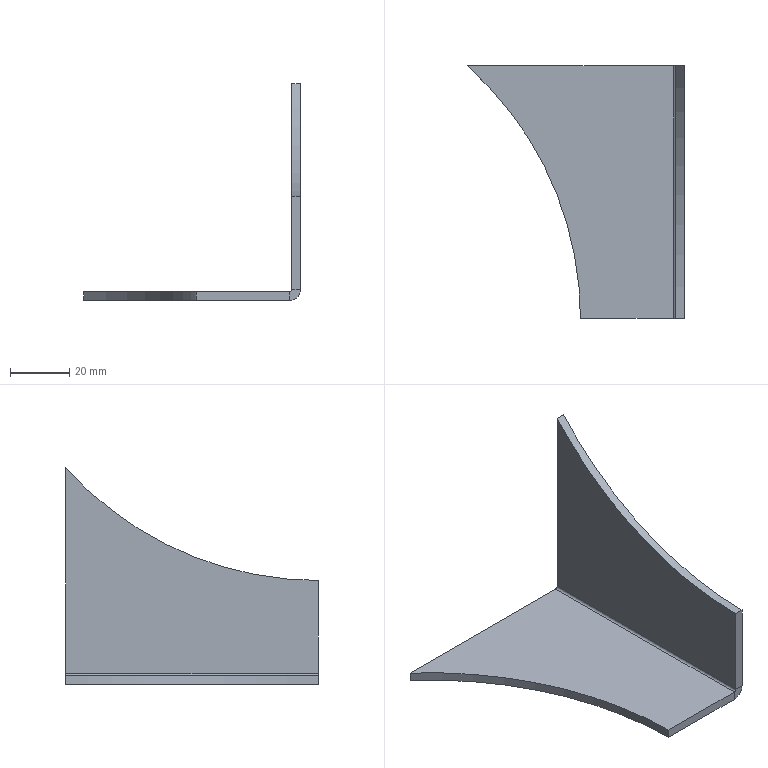Component | SolidWorks | CCQ-1.1-21SupportBendPart-2 | 1 solid | 14 faces | box 73 x 85 x 73 mm | volume 22798 mm3 | plane 10 | cylinder 4 | commonest cylinder face diameters 228.132 x2 1.473 x1 7.473 x1 | material 304
STEP:
#1=CARTESIAN_POINT('',(1.428,-21.398,-16.024));
#2=VERTEX_POINT('',#1);
#3=CARTESIAN_POINT('',(0.1969,-21.398,-16.024));
#4=VERTEX_POINT('',#3);
#5=CARTESIAN_POINT('',(1.457,-21.398,-16.024));
#6=DIRECTION('',(-1.,-0.,0.));
#7=VECTOR('',#6,39.37);
#8=LINE('',#5,#7);
#9=EDGE_CURVE('',#2,#4,#8,.T.);
#10=ORIENTED_EDGE('',*,*,#9,.T.);
#11=CARTESIAN_POINT('',(0.1969,-21.398,-16.142));
#12=VERTEX_POINT('',#11);
#13=CARTESIAN_POINT('',(0.1969,-21.398,-16.024));
#14=DIRECTION('',(-0.,0.,-1.));
#15=VECTOR('',#14,39.37);
#16=LINE('',#13,#15);
#17=EDGE_CURVE('',#4,#12,#16,.T.);
#18=ORIENTED_EDGE('',*,*,#17,.T.);
#19=CARTESIAN_POINT('',(1.428,-21.398,-16.142));
#20=VERTEX_POINT('',#19);
#21=CARTESIAN_POINT('',(1.457,-21.398,-16.142));
#22=DIRECTION('',(-1.,-0.,0.));
#23=VECTOR('',#22,39.37);
#24=LINE('',#21,#23);
#25=EDGE_CURVE('',#20,#12,#24,.T.);
#26=ORIENTED_EDGE('',*,*,#25,.F.);
#27=CARTESIAN_POINT('',(1.428,-21.398,-16.142));
#28=DIRECTION('',(0.,-0.,1.));
#29=VECTOR('',#28,39.37);
#30=LINE('',#27,#29);
#31=EDGE_CURVE('',#20,#2,#30,.T.);
#32=ORIENTED_EDGE('',*,*,#31,.T.);
#33=EDGE_LOOP('',(#10,#18,#26,#32));
#34=FACE_OUTER_BOUND('',#33,.T.);
#35=CARTESIAN_POINT('',(1.428,-21.398,-15.995));
#36=DIRECTION('',(0.,-1.,-0.));
#37=DIRECTION('',(0.,0.,-1.));
#38=AXIS2_PLACEMENT_3D('',#35,#36,#37);
#39=PLANE('',#38);
#40=ADVANCED_FACE('',(#34),#39,.T.);
#41=CARTESIAN_POINT('',(1.428,-18.051,-16.024));
#42=VERTEX_POINT('',#41);
#43=CARTESIAN_POINT('',(1.428,-18.051,-16.142));
#44=VERTEX_POINT('',#43);
#45=CARTESIAN_POINT('',(1.428,-18.051,-16.024));
#46=DIRECTION('',(-0.,0.,-1.));
#47=VECTOR('',#46,39.37);
#48=LINE('',#45,#47);
#49=EDGE_CURVE('',#42,#44,#48,.T.);
#50=ORIENTED_EDGE('',*,*,#49,.F.);
#51=CARTESIAN_POINT('',(1.457,-18.051,-15.995));
#52=VERTEX_POINT('',#51);
#53=CARTESIAN_POINT('',(1.428,-18.051,-15.995));
#54=DIRECTION('',(-0.,1.,0.));
#55=DIRECTION('',(1.,0.,0.));
#56=AXIS2_PLACEMENT_3D('',#53,#54,#55);
#57=CIRCLE('',#56,0.029);
#58=EDGE_CURVE('',#52,#42,#57,.T.);
#59=ORIENTED_EDGE('',*,*,#58,.F.);
#60=CARTESIAN_POINT('',(1.575,-18.051,-15.995));
#61=VERTEX_POINT('',#60);
#62=CARTESIAN_POINT('',(1.575,-18.051,-15.995));
#63=DIRECTION('',(-1.,-0.,-0.));
#64=VECTOR('',#63,39.37);
#65=LINE('',#62,#64);
#66=EDGE_CURVE('',#61,#52,#65,.T.);
#67=ORIENTED_EDGE('',*,*,#66,.F.);
#68=CARTESIAN_POINT('',(1.428,-18.051,-15.995));
#69=DIRECTION('',(-0.,1.,0.));
#70=DIRECTION('',(0.,0.,1.));
#71=AXIS2_PLACEMENT_3D('',#68,#69,#70);
#72=CIRCLE('',#71,0.1471);
#73=EDGE_CURVE('',#61,#44,#72,.T.);
#74=ORIENTED_EDGE('',*,*,#73,.T.);
#75=EDGE_LOOP('',(#50,#59,#67,#74));
#76=FACE_OUTER_BOUND('',#75,.T.);
#77=CARTESIAN_POINT('',(1.428,-18.051,-16.024));
#78=DIRECTION('',(-0.,1.,0.));
#79=DIRECTION('',(-1.,-0.,0.));
#80=AXIS2_PLACEMENT_3D('',#77,#78,#79);
#81=PLANE('',#80);
#82=ADVANCED_FACE('',(#76),#81,.T.);
#83=CARTESIAN_POINT('',(-1.299,-18.051,-16.024));
#84=VERTEX_POINT('',#83);
#85=CARTESIAN_POINT('',(1.457,-18.051,-16.024));
#86=DIRECTION('',(-1.,-0.,0.));
#87=VECTOR('',#86,39.37);
#88=LINE('',#85,#87);
#89=EDGE_CURVE('',#42,#84,#88,.T.);
#90=ORIENTED_EDGE('',*,*,#89,.F.);
#91=ORIENTED_EDGE('',*,*,#49,.T.);
#92=CARTESIAN_POINT('',(-1.299,-18.051,-16.142));
#93=VERTEX_POINT('',#92);
#94=CARTESIAN_POINT('',(1.457,-18.051,-16.142));
#95=DIRECTION('',(-1.,-0.,0.));
#96=VECTOR('',#95,39.37);
#97=LINE('',#94,#96);
#98=EDGE_CURVE('',#44,#93,#97,.T.);
#99=ORIENTED_EDGE('',*,*,#98,.T.);
#100=CARTESIAN_POINT('',(-1.299,-18.051,-16.024));
#101=DIRECTION('',(0.,0.,-1.));
#102=VECTOR('',#101,39.37);
#103=LINE('',#100,#102);
#104=EDGE_CURVE('',#84,#93,#103,.T.);
#105=ORIENTED_EDGE('',*,*,#104,.F.);
#106=EDGE_LOOP('',(#90,#91,#99,#105));
#107=FACE_OUTER_BOUND('',#106,.T.);
#108=CARTESIAN_POINT('',(1.575,-18.051,-15.995));
#109=DIRECTION('',(-0.,1.,0.));
#110=DIRECTION('',(-1.,-0.,0.));
#111=AXIS2_PLACEMENT_3D('',#108,#109,#110);
#112=PLANE('',#111);
#113=ADVANCED_FACE('',(#107),#112,.T.);
#114=CARTESIAN_POINT('',(1.457,-21.398,-15.995));
#115=VERTEX_POINT('',#114);
#116=CARTESIAN_POINT('',(1.575,-21.398,-15.995));
#117=VERTEX_POINT('',#116);
#118=CARTESIAN_POINT('',(1.457,-21.398,-15.995));
#119=DIRECTION('',(1.,0.,0.));
#120=VECTOR('',#119,39.37);
#121=LINE('',#118,#120);
#122=EDGE_CURVE('',#115,#117,#121,.T.);
#123=ORIENTED_EDGE('',*,*,#122,.F.);
#124=CARTESIAN_POINT('',(1.428,-21.398,-15.995));
#125=DIRECTION('',(-0.,1.,0.));
#126=DIRECTION('',(1.,0.,0.));
#127=AXIS2_PLACEMENT_3D('',#124,#125,#126);
#128=CIRCLE('',#127,0.029);
#129=EDGE_CURVE('',#115,#2,#128,.T.);
#130=ORIENTED_EDGE('',*,*,#129,.T.);
#131=ORIENTED_EDGE('',*,*,#31,.F.);
#132=CARTESIAN_POINT('',(1.428,-21.398,-15.995));
#133=DIRECTION('',(-0.,1.,0.));
#134=DIRECTION('',(0.,0.,1.));
#135=AXIS2_PLACEMENT_3D('',#132,#133,#134);
#136=CIRCLE('',#135,0.1471);
#137=EDGE_CURVE('',#117,#20,#136,.T.);
#138=ORIENTED_EDGE('',*,*,#137,.F.);
#139=EDGE_LOOP('',(#123,#130,#131,#138));
#140=FACE_OUTER_BOUND('',#139,.T.);
#141=CARTESIAN_POINT('',(1.457,-21.398,-15.995));
#142=DIRECTION('',(0.,-1.,-0.));
#143=DIRECTION('',(1.,0.,-0.));
#144=AXIS2_PLACEMENT_3D('',#141,#142,#143);
#145=PLANE('',#144);
#146=ADVANCED_FACE('',(#140),#145,.T.);
#147=CARTESIAN_POINT('',(1.457,-21.398,-14.764));
#148=VERTEX_POINT('',#147);
#149=CARTESIAN_POINT('',(1.575,-21.398,-14.764));
#150=VERTEX_POINT('',#149);
#151=CARTESIAN_POINT('',(1.181,-21.398,-14.764));
#152=DIRECTION('',(1.,0.,-0.));
#153=VECTOR('',#152,39.37);
#154=LINE('',#151,#153);
#155=EDGE_CURVE('',#148,#150,#154,.T.);
#156=ORIENTED_EDGE('',*,*,#155,.F.);
#157=CARTESIAN_POINT('',(1.457,-21.398,-16.024));
#158=DIRECTION('',(0.,0.,-1.));
#159=VECTOR('',#158,39.37);
#160=LINE('',#157,#159);
#161=EDGE_CURVE('',#148,#115,#160,.T.);
#162=ORIENTED_EDGE('',*,*,#161,.T.);
#163=ORIENTED_EDGE('',*,*,#122,.T.);
#164=CARTESIAN_POINT('',(1.575,-21.398,-16.024));
#165=DIRECTION('',(0.,0.,-1.));
#166=VECTOR('',#165,39.37);
#167=LINE('',#164,#166);
#168=EDGE_CURVE('',#150,#117,#167,.T.);
#169=ORIENTED_EDGE('',*,*,#168,.F.);
#170=EDGE_LOOP('',(#156,#162,#163,#169));
#171=FACE_OUTER_BOUND('',#170,.T.);
#172=CARTESIAN_POINT('',(1.428,-21.398,-16.142));
#173=DIRECTION('',(0.,-1.,-0.));
#174=DIRECTION('',(1.,0.,-0.));
#175=AXIS2_PLACEMENT_3D('',#172,#173,#174);
#176=PLANE('',#175);
#177=ADVANCED_FACE('',(#171),#176,.T.);
#178=CARTESIAN_POINT('',(-4.294,-21.398,-16.142));
#179=DIRECTION('',(0.,-0.,1.));
#180=DIRECTION('',(1.,0.,0.));
#181=AXIS2_PLACEMENT_3D('',#178,#179,#180);
#182=CIRCLE('',#181,4.491);
#183=EDGE_CURVE('',#12,#93,#182,.T.);
#184=ORIENTED_EDGE('',*,*,#183,.T.);
#185=ORIENTED_EDGE('',*,*,#98,.F.);
#186=CARTESIAN_POINT('',(1.428,-18.051,-16.142));
#187=DIRECTION('',(0.,-1.,-0.));
#188=VECTOR('',#187,39.37);
#189=LINE('',#186,#188);
#190=EDGE_CURVE('',#44,#20,#189,.T.);
#191=ORIENTED_EDGE('',*,*,#190,.T.);
#192=ORIENTED_EDGE('',*,*,#25,.T.);
#193=EDGE_LOOP('',(#184,#185,#191,#192));
#194=FACE_OUTER_BOUND('',#193,.T.);
#195=CARTESIAN_POINT('',(1.457,-18.051,-16.142));
#196=DIRECTION('',(0.,-0.,1.));
#197=DIRECTION('',(1.,0.,-0.));
#198=AXIS2_PLACEMENT_3D('',#195,#196,#197);
#199=PLANE('',#198);
#200=ADVANCED_FACE('',(#194),#199,.F.);
#201=ORIENTED_EDGE('',*,*,#89,.T.);
#202=CARTESIAN_POINT('',(-4.294,-21.398,-16.024));
#203=DIRECTION('',(0.,-0.,1.));
#204=DIRECTION('',(1.,0.,0.));
#205=AXIS2_PLACEMENT_3D('',#202,#203,#204);
#206=CIRCLE('',#205,4.491);
#207=EDGE_CURVE('',#4,#84,#206,.T.);
#208=ORIENTED_EDGE('',*,*,#207,.F.);
#209=ORIENTED_EDGE('',*,*,#9,.F.);
#210=CARTESIAN_POINT('',(1.428,-18.051,-16.024));
#211=DIRECTION('',(0.,-1.,-0.));
#212=VECTOR('',#211,39.37);
#213=LINE('',#210,#212);
#214=EDGE_CURVE('',#42,#2,#213,.T.);
#215=ORIENTED_EDGE('',*,*,#214,.F.);
#216=EDGE_LOOP('',(#201,#208,#209,#215));
#217=FACE_OUTER_BOUND('',#216,.T.);
#218=CARTESIAN_POINT('',(1.457,-18.051,-16.024));
#219=DIRECTION('',(0.,-0.,1.));
#220=DIRECTION('',(1.,0.,-0.));
#221=AXIS2_PLACEMENT_3D('',#218,#219,#220);
#222=PLANE('',#221);
#223=ADVANCED_FACE('',(#217),#222,.T.);
#224=ORIENTED_EDGE('',*,*,#129,.F.);
#225=CARTESIAN_POINT('',(1.457,-18.051,-15.995));
#226=DIRECTION('',(0.,-1.,-0.));
#227=VECTOR('',#226,39.37);
#228=LINE('',#225,#227);
#229=EDGE_CURVE('',#52,#115,#228,.T.);
#230=ORIENTED_EDGE('',*,*,#229,.F.);
#231=ORIENTED_EDGE('',*,*,#58,.T.);
#232=ORIENTED_EDGE('',*,*,#214,.T.);
#233=EDGE_LOOP('',(#224,#230,#231,#232));
#234=FACE_OUTER_BOUND('',#233,.T.);
#235=CARTESIAN_POINT('',(1.428,-18.051,-15.995));
#236=DIRECTION('',(0.,-1.,-0.));
#237=DIRECTION('',(1.,0.,0.));
#238=AXIS2_PLACEMENT_3D('',#235,#236,#237);
#239=CYLINDRICAL_SURFACE('',#238,0.029);
#240=ADVANCED_FACE('',(#234),#239,.F.);
#241=CARTESIAN_POINT('',(1.457,-18.051,-13.268));
#242=VERTEX_POINT('',#241);
#243=CARTESIAN_POINT('',(1.457,-21.398,-10.273));
#244=DIRECTION('',(-1.,-0.,0.));
#245=DIRECTION('',(-0.,0.,1.));
#246=AXIS2_PLACEMENT_3D('',#243,#244,#245);
#247=CIRCLE('',#246,4.491);
#248=EDGE_CURVE('',#242,#148,#247,.T.);
#249=ORIENTED_EDGE('',*,*,#248,.F.);
#250=CARTESIAN_POINT('',(1.457,-18.051,-16.024));
#251=DIRECTION('',(0.,0.,-1.));
#252=VECTOR('',#251,39.37);
#253=LINE('',#250,#252);
#254=EDGE_CURVE('',#242,#52,#253,.T.);
#255=ORIENTED_EDGE('',*,*,#254,.T.);
#256=ORIENTED_EDGE('',*,*,#229,.T.);
#257=ORIENTED_EDGE('',*,*,#161,.F.);
#258=EDGE_LOOP('',(#249,#255,#256,#257));
#259=FACE_OUTER_BOUND('',#258,.T.);
#260=CARTESIAN_POINT('',(1.457,-18.051,-16.024));
#261=DIRECTION('',(-1.,-0.,-0.));
#262=DIRECTION('',(-0.,-0.,1.));
#263=AXIS2_PLACEMENT_3D('',#260,#261,#262);
#264=PLANE('',#263);
#265=ADVANCED_FACE('',(#259),#264,.T.);
#266=CARTESIAN_POINT('',(1.575,-18.051,-13.268));
#267=VERTEX_POINT('',#266);
#268=CARTESIAN_POINT('',(1.575,-18.051,-16.024));
#269=DIRECTION('',(0.,0.,-1.));
#270=VECTOR('',#269,39.37);
#271=LINE('',#268,#270);
#272=EDGE_CURVE('',#267,#61,#271,.T.);
#273=ORIENTED_EDGE('',*,*,#272,.F.);
#274=CARTESIAN_POINT('',(1.575,-21.398,-10.273));
#275=DIRECTION('',(1.,0.,-0.));
#276=DIRECTION('',(-0.,0.,1.));
#277=AXIS2_PLACEMENT_3D('',#274,#275,#276);
#278=CIRCLE('',#277,4.491);
#279=EDGE_CURVE('',#150,#267,#278,.T.);
#280=ORIENTED_EDGE('',*,*,#279,.F.);
#281=ORIENTED_EDGE('',*,*,#168,.T.);
#282=CARTESIAN_POINT('',(1.575,-18.051,-15.995));
#283=DIRECTION('',(0.,-1.,-0.));
#284=VECTOR('',#283,39.37);
#285=LINE('',#282,#284);
#286=EDGE_CURVE('',#61,#117,#285,.T.);
#287=ORIENTED_EDGE('',*,*,#286,.F.);
#288=EDGE_LOOP('',(#273,#280,#281,#287));
#289=FACE_OUTER_BOUND('',#288,.T.);
#290=CARTESIAN_POINT('',(1.575,-18.051,-16.024));
#291=DIRECTION('',(-1.,-0.,-0.));
#292=DIRECTION('',(-0.,-0.,1.));
#293=AXIS2_PLACEMENT_3D('',#290,#291,#292);
#294=PLANE('',#293);
#295=ADVANCED_FACE('',(#289),#294,.F.);
#296=ORIENTED_EDGE('',*,*,#137,.T.);
#297=ORIENTED_EDGE('',*,*,#190,.F.);
#298=ORIENTED_EDGE('',*,*,#73,.F.);
#299=ORIENTED_EDGE('',*,*,#286,.T.);
#300=EDGE_LOOP('',(#296,#297,#298,#299));
#301=FACE_OUTER_BOUND('',#300,.T.);
#302=CARTESIAN_POINT('',(1.428,-18.051,-15.995));
#303=DIRECTION('',(0.,-1.,-0.));
#304=DIRECTION('',(1.,0.,0.));
#305=AXIS2_PLACEMENT_3D('',#302,#303,#304);
#306=CYLINDRICAL_SURFACE('',#305,0.1471);
#307=ADVANCED_FACE('',(#301),#306,.T.);
#308=ORIENTED_EDGE('',*,*,#272,.T.);
#309=ORIENTED_EDGE('',*,*,#66,.T.);
#310=ORIENTED_EDGE('',*,*,#254,.F.);
#311=CARTESIAN_POINT('',(1.575,-18.051,-13.268));
#312=DIRECTION('',(-1.,-0.,0.));
#313=VECTOR('',#312,39.37);
#314=LINE('',#311,#313);
#315=EDGE_CURVE('',#267,#242,#314,.T.);
#316=ORIENTED_EDGE('',*,*,#315,.F.);
#317=EDGE_LOOP('',(#308,#309,#310,#316));
#318=FACE_OUTER_BOUND('',#317,.T.);
#319=CARTESIAN_POINT('',(1.428,-18.051,-15.995));
#320=DIRECTION('',(0.,-1.,-0.));
#321=DIRECTION('',(0.,0.,-1.));
#322=AXIS2_PLACEMENT_3D('',#319,#320,#321);
#323=PLANE('',#322);
#324=ADVANCED_FACE('',(#318),#323,.F.);
#325=ORIENTED_EDGE('',*,*,#207,.T.);
#326=ORIENTED_EDGE('',*,*,#104,.T.);
#327=ORIENTED_EDGE('',*,*,#183,.F.);
#328=ORIENTED_EDGE('',*,*,#17,.F.);
#329=EDGE_LOOP('',(#325,#326,#327,#328));
#330=FACE_OUTER_BOUND('',#329,.T.);
#331=CARTESIAN_POINT('',(-4.294,-21.398,-16.024));
#332=DIRECTION('',(0.,-0.,1.));
#333=DIRECTION('',(1.,0.,0.));
#334=AXIS2_PLACEMENT_3D('',#331,#332,#333);
#335=CYLINDRICAL_SURFACE('',#334,4.491);
#336=ADVANCED_FACE('',(#330),#335,.F.);
#337=ORIENTED_EDGE('',*,*,#248,.T.);
#338=ORIENTED_EDGE('',*,*,#155,.T.);
#339=ORIENTED_EDGE('',*,*,#279,.T.);
#340=ORIENTED_EDGE('',*,*,#315,.T.);
#341=EDGE_LOOP('',(#337,#338,#339,#340));
#342=FACE_OUTER_BOUND('',#341,.T.);
#343=CARTESIAN_POINT('',(1.181,-21.398,-10.273));
#344=DIRECTION('',(1.,0.,-0.));
#345=DIRECTION('',(0.,0.,-1.));
#346=AXIS2_PLACEMENT_3D('',#343,#344,#345);
#347=CYLINDRICAL_SURFACE('',#346,4.491);
#348=ADVANCED_FACE('',(#342),#347,.F.);
#349=CLOSED_SHELL('',(#40,#82,#113,#146,#177,#200,#223,#240,#265,#295,#307,#324,#336,#348));
#350=MANIFOLD_SOLID_BREP('',#349);
#351=CARTESIAN_POINT('',(0.,0.,0.));
#352=DIRECTION('',(0.,0.,1.));
#353=DIRECTION('',(1.,0.,0.));
#354=AXIS2_PLACEMENT_3D('',#351,#352,#353);
#355=(LENGTH_UNIT()NAMED_UNIT(*)SI_UNIT($,.METRE.));
#356=LENGTH_MEASURE_WITH_UNIT(LENGTH_MEASURE(0.0254),#355);
#357=DIMENSIONAL_EXPONENTS(1.,0.,0.,0.,0.,0.,0.);
#358=(CONVERSION_BASED_UNIT('',#356)LENGTH_UNIT()NAMED_UNIT(#357));
#359=UNCERTAINTY_MEASURE_WITH_UNIT(LENGTH_MEASURE(0.00001),#358,'','');
#360=(NAMED_UNIT(*)PLANE_ANGLE_UNIT()SI_UNIT($,.RADIAN.));
#361=(NAMED_UNIT(*)SI_UNIT($,.STERADIAN.)SOLID_ANGLE_UNIT());
#362=(GEOMETRIC_REPRESENTATION_CONTEXT(3)GLOBAL_UNCERTAINTY_ASSIGNED_CONTEXT((#359))GLOBAL_UNIT_ASSIGNED_CONTEXT((#358,#360,#361))REPRESENTATION_CONTEXT('',''));
#363=ADVANCED_BREP_SHAPE_REPRESENTATION('',(#350,#354),#362);
#364=COLOUR_RGB('',0.7922,0.8196,0.9333);
#365=FILL_AREA_STYLE_COLOUR('',#364);
#366=FILL_AREA_STYLE('',(#365));
#367=SURFACE_STYLE_FILL_AREA(#366);
#368=SURFACE_SIDE_STYLE('',(#367));
#369=SURFACE_STYLE_USAGE(.BOTH.,#368);
#370=PRESENTATION_STYLE_ASSIGNMENT((#369));
#371=STYLED_ITEM('',(#370),#350);
#372=(LENGTH_UNIT()NAMED_UNIT(*)SI_UNIT($,.METRE.));
#373=LENGTH_MEASURE_WITH_UNIT(LENGTH_MEASURE(0.0254),#372);
#374=DIMENSIONAL_EXPONENTS(1.,0.,0.,0.,0.,0.,0.);
#375=(CONVERSION_BASED_UNIT('',#373)LENGTH_UNIT()NAMED_UNIT(#374));
#376=UNCERTAINTY_MEASURE_WITH_UNIT(LENGTH_MEASURE(0.00001),#375,'','');
#377=(NAMED_UNIT(*)PLANE_ANGLE_UNIT()SI_UNIT($,.RADIAN.));
#378=(NAMED_UNIT(*)SI_UNIT($,.STERADIAN.)SOLID_ANGLE_UNIT());
#379=(GEOMETRIC_REPRESENTATION_CONTEXT(3)GLOBAL_UNCERTAINTY_ASSIGNED_CONTEXT((#376))GLOBAL_UNIT_ASSIGNED_CONTEXT((#375,#377,#378))REPRESENTATION_CONTEXT('',''));
#380=MECHANICAL_DESIGN_GEOMETRIC_PRESENTATION_REPRESENTATION('',(#371),#379);
#381=PRESENTATION_LAYER_ASSIGNMENT('','',(#371));